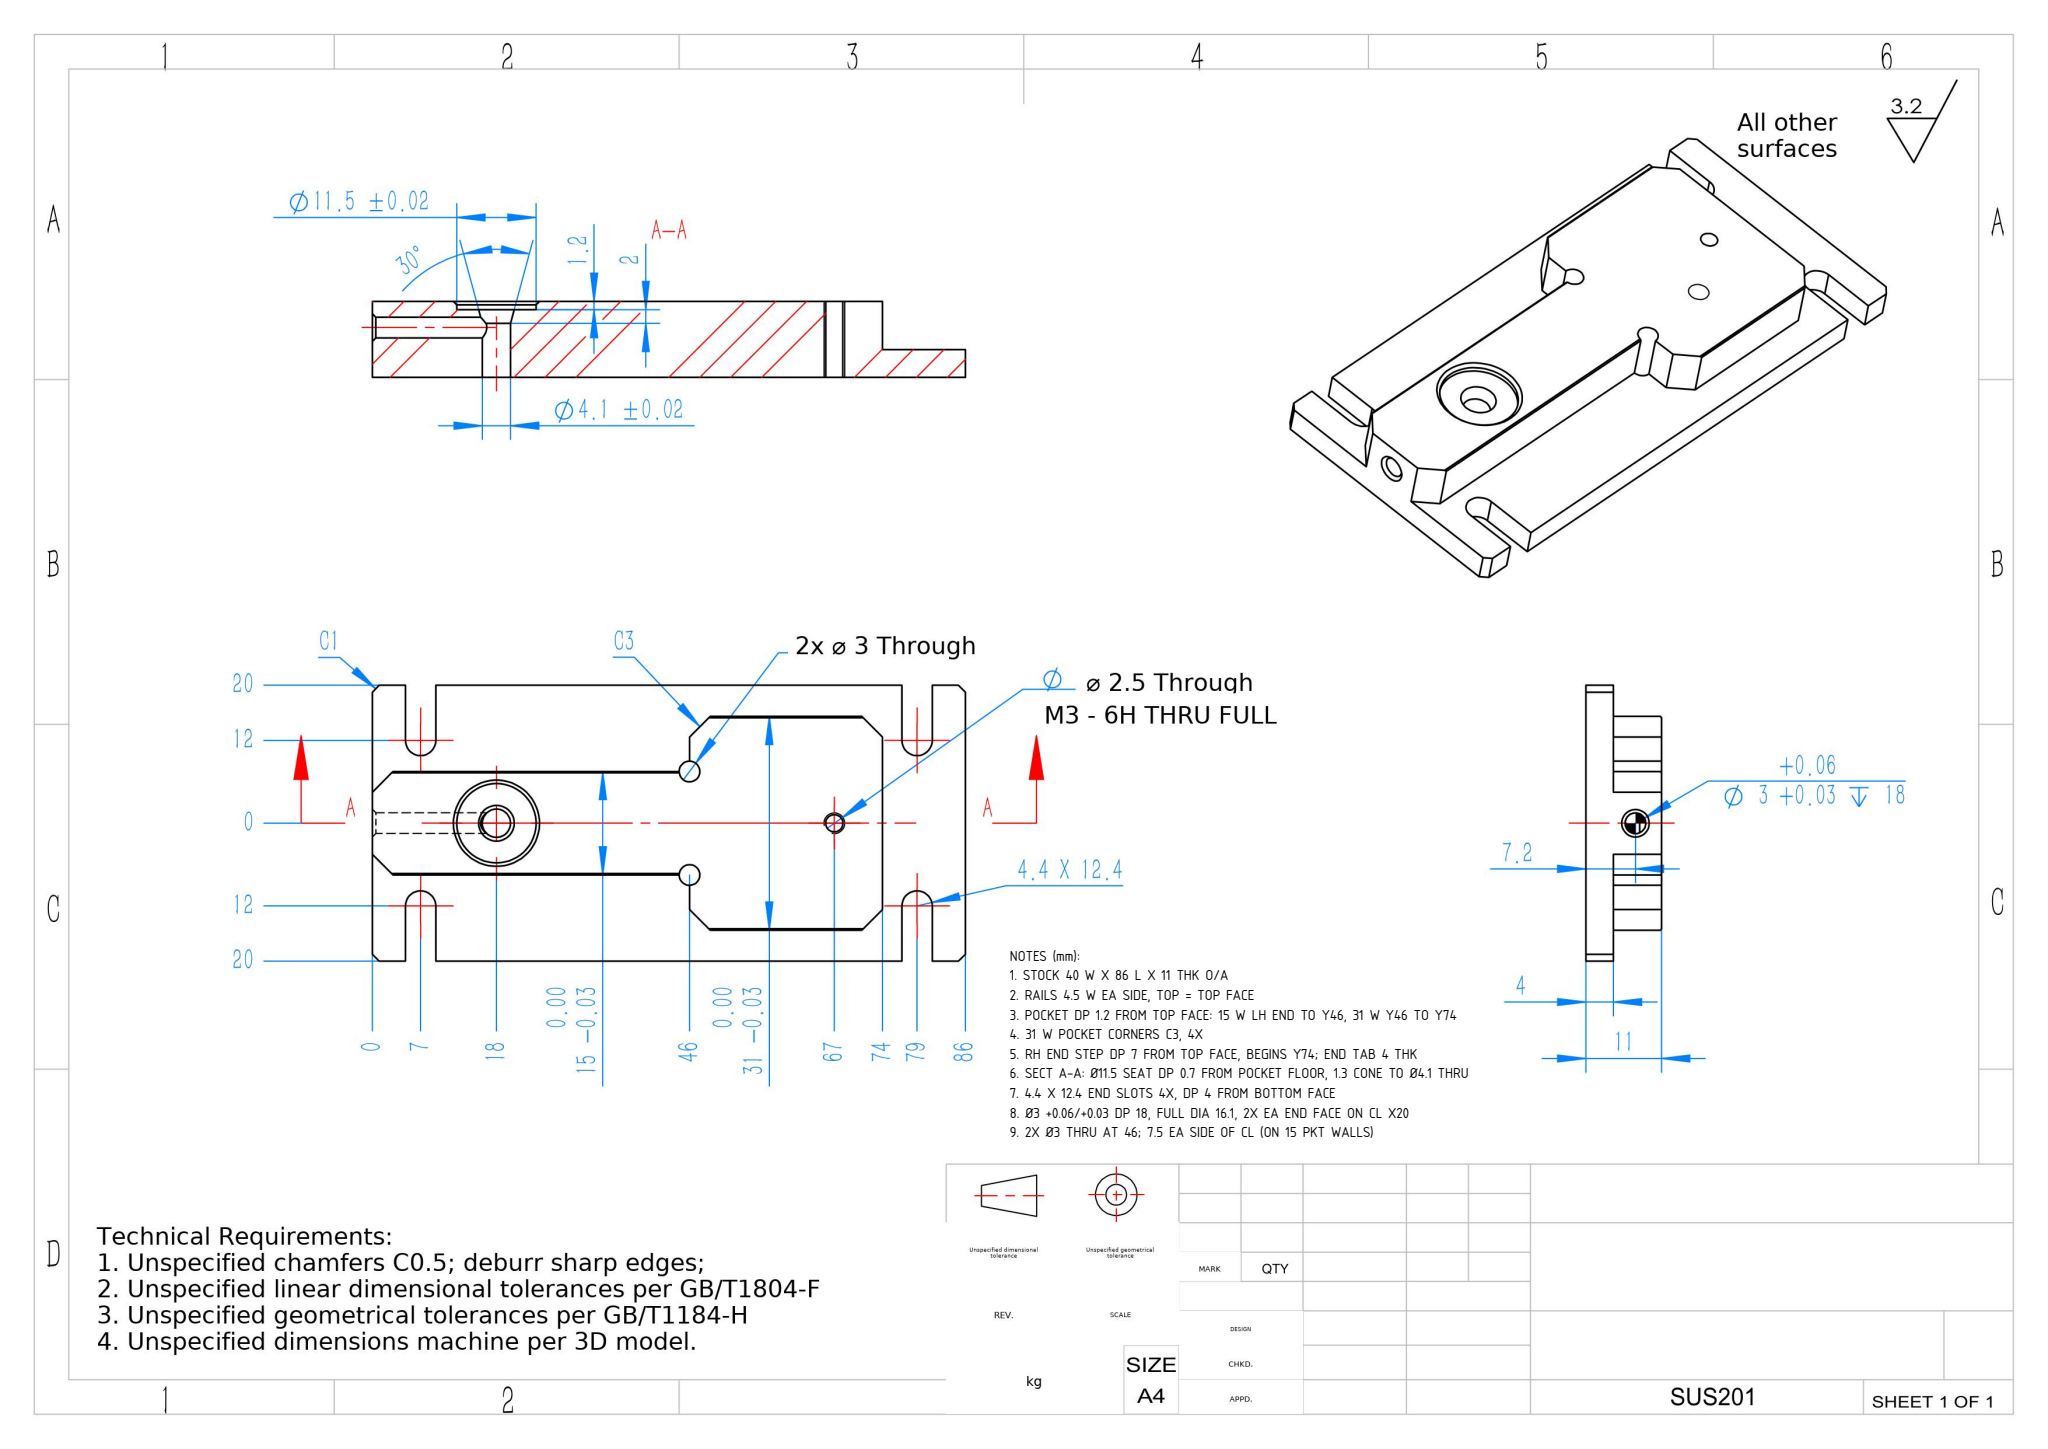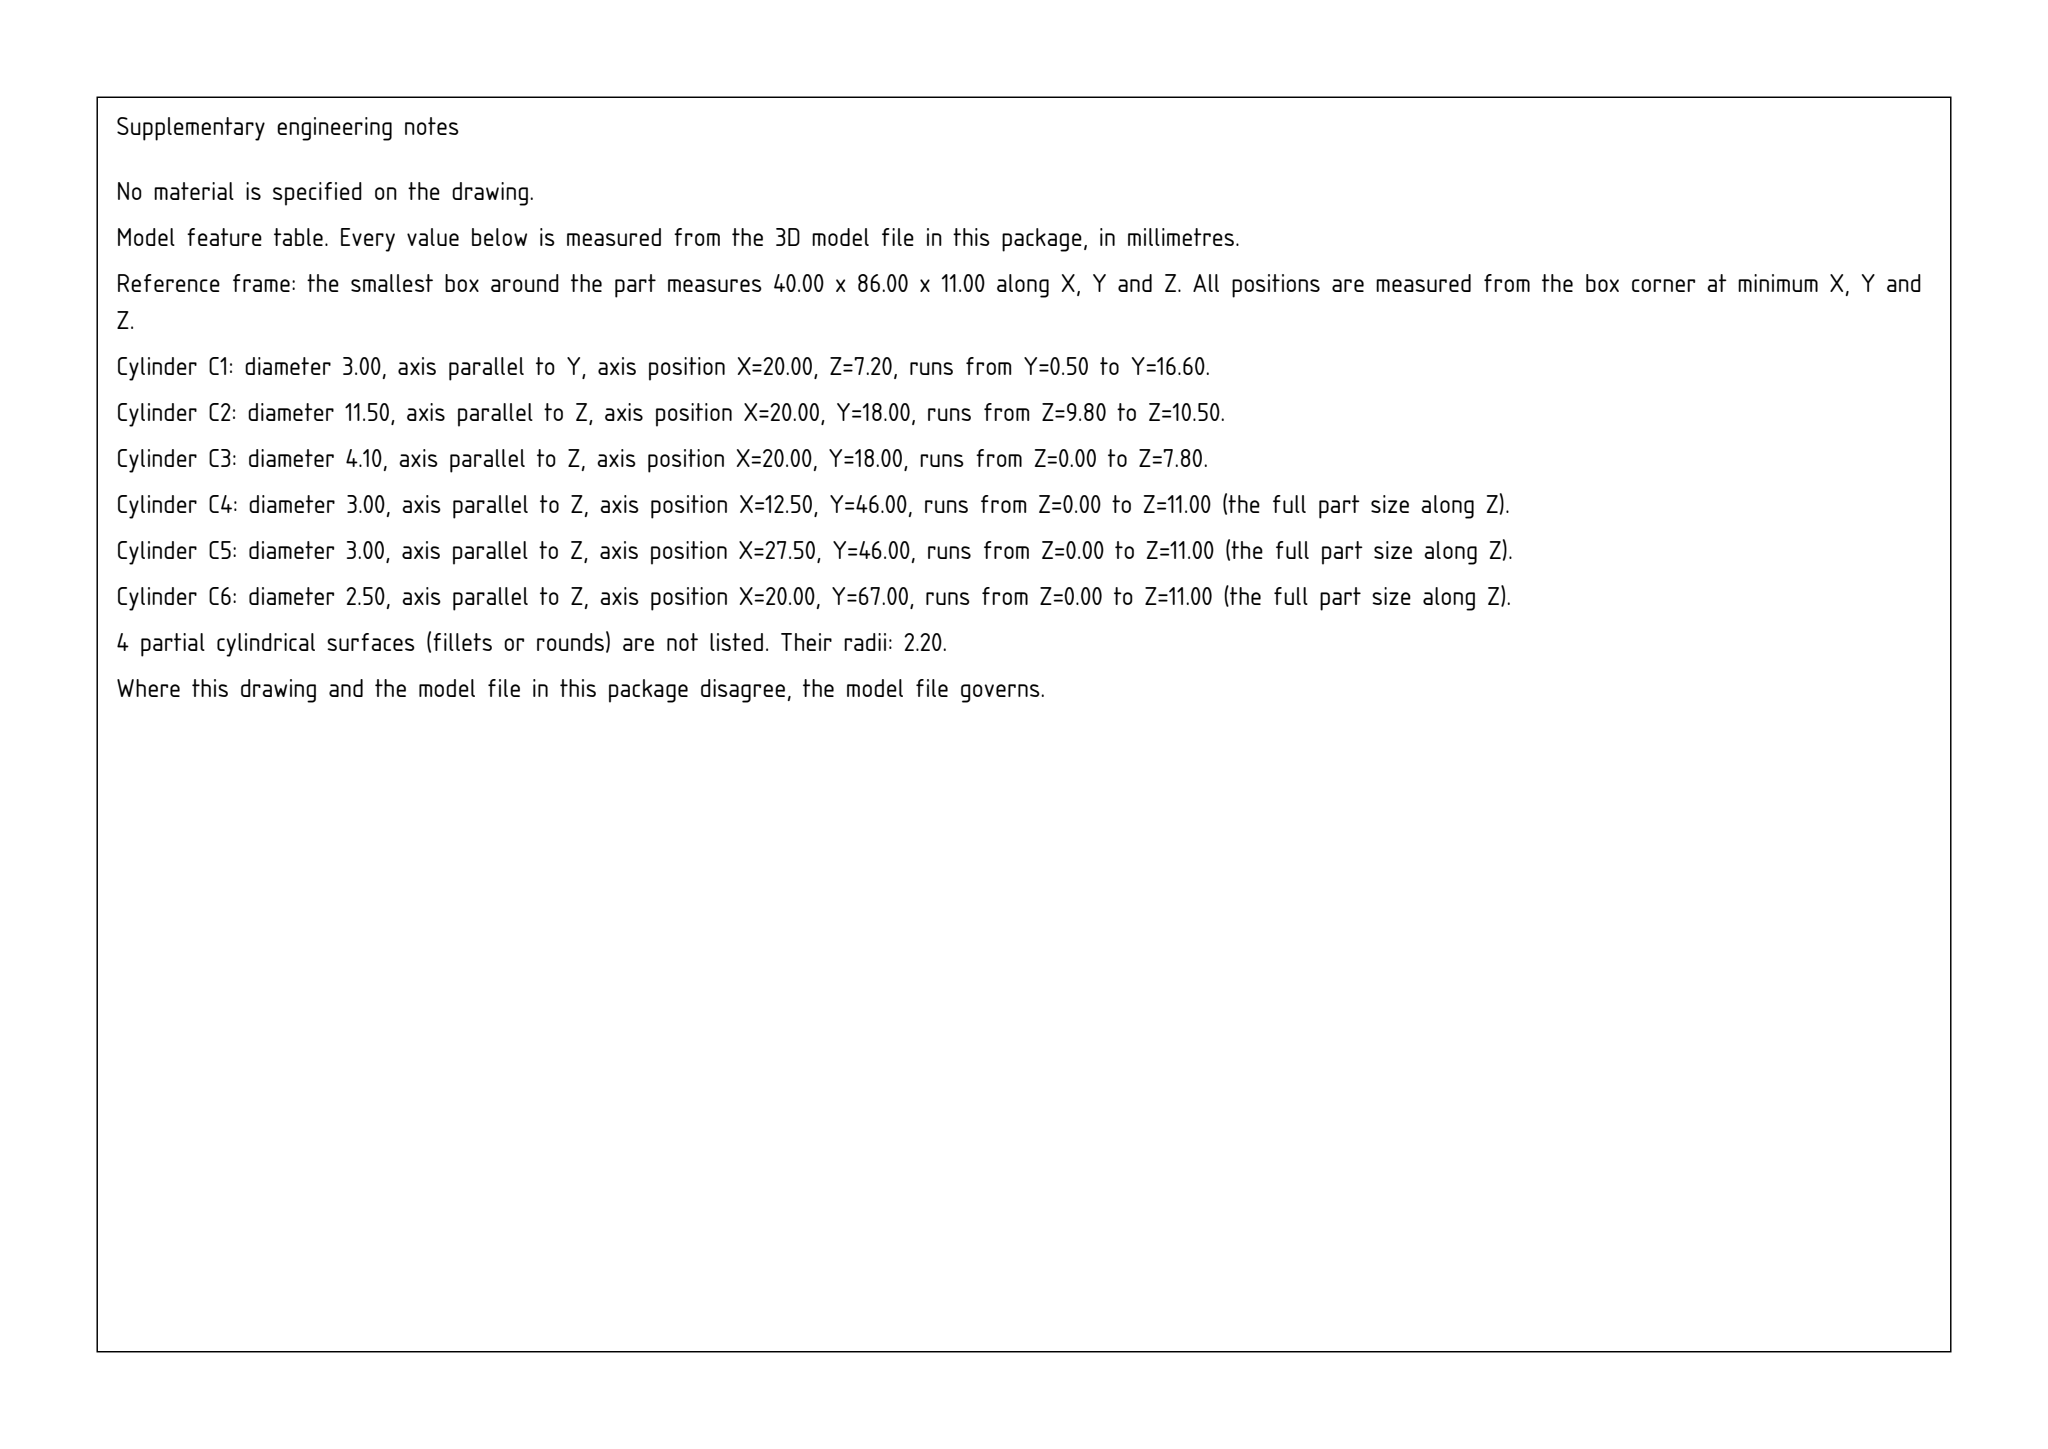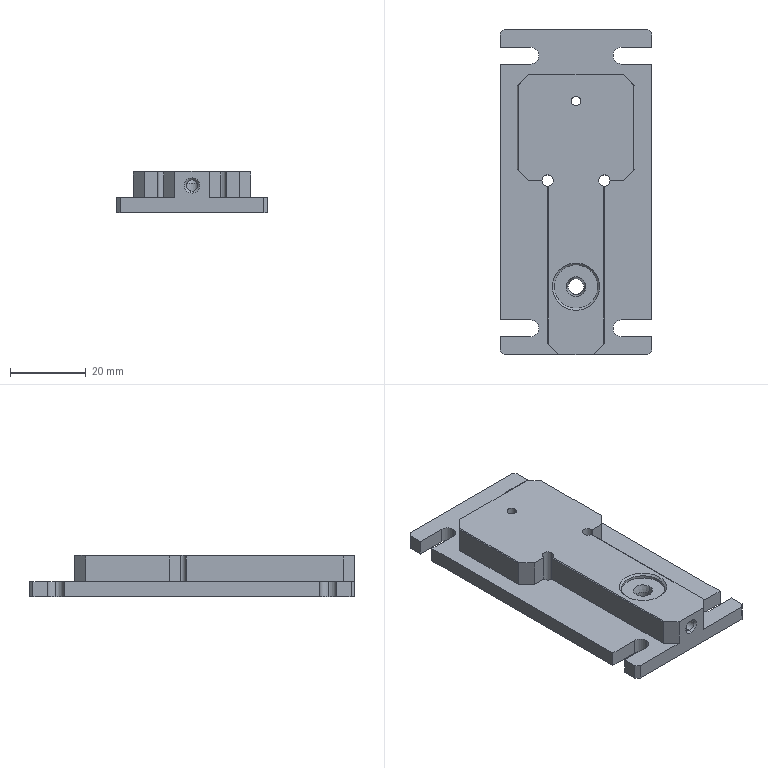Part | SolidWorks | mm | 1 solid | 65 faces | box 40 x 86 x 11 mm | volume 23216 mm3 | plane 41 | cylinder 18 | cone 6 | commonest cylinder face diameters 4.4 x6 3 x6 2.5 x2 4.1 x2 11.5 x2
Drawing notes:
STOCK 40 W X 86 L X 11 THK O/A | from the solid: bbox_xyz 40 x 86 x 11
RAILS 4.5 W EA SIDE, TOP = TOP FACE | from the solid: x-planes 0/4.5 and 35.5/40
POCKET DP 1.2 FROM TOP FACE: 15 W LH END TO Y46, 31 W Y46 TO Y74 | from the solid: z-plane 9.8 vs top 11.0; x 12.5/27.5 (15 W), x 4.5/35.5 (31 W); y 0/46/74
31 W POCKET CORNERS C3, 4X | from the solid: no fillet_radii; 45° corner reliefs at x4.5/35.5, y46/74
RH END STEP DP 7 FROM TOP FACE, BEGINS Y74; END TAB 4 THK | from the solid: y-plane 74.0; step face z=4.0 vs top z=11.0; tab z0-4 to y=86
SECT A-A: Ø11.5 SEAT DP 0.7 FROM POCKET FLOOR, 1.3 CONE TO Ø4.1 THRU | from the solid: Ø11.5 len 0.7 at (20,18); floor z=9.8; Ø4.1 len 7.8 to z=0; 9.8-0.7-7.8=1.3
4.4 X 12.4 END SLOTS 4X, DP 4 FROM BOTTOM FACE | from the solid: Ø4.4 z-cyls at (8,7),(32,7),(8,79),(32,79) len 4.0 from z=0; z-plane 4.0
Ø3 +0.06/+0.03 DP 18, FULL DIA 16.1, 2X EA END FACE ON CL X20 | from the solid: cyl [3.0,'y',x=20,z=7.2,len 16.1,qty 2] + 90° drill point; bbox X=40
2X Ø3 THRU AT 46; 7.5 EA SIDE OF CL (ON 15 PKT WALLS) | from the solid: cylinders dia 3.0 axis z at (12.5,46) and (27.5,46), length 11 = full thk; part CL at x=20, bbox 40x86x11
build123d program:
from build123d import *

# Parameters (mm, degrees)
SKETCH1_W                      = 15
SKETCH1_H                      = 86
BOSS_EXTRUDE1_DEPTH            = 11
SKETCH14_W                     = 40
SKETCH14_H                     = 86
BOSS_EXTRUDE3_DEPTH            = 4
SKETCH3_R                      = 5.75
CUT_EXTRUDE2_DEPTH             = 1.2
F_5_2_5_2_DIAMETER_HOLE1_D     = 4.1
CHAMFER1_SIZE                  = 0.5
CHAMFER2_SIZE                  = 2
CHAMFER2_SIZE2                 = 0.5359
M3_TAPPED_HOLE1_D              = 2.5
SIZE_MM_DOWEL_PIN_HOLE_1_D     = 3
SIZE_MM_DOWEL_PIN_HOLE_1_DEPTH = 18
SIZE_MM_DOWEL_PIN_HOLE_1_TIP   = 0.9013
CHAMFER3_SIZE                  = 0.5
F_4_0_4_DIAMETER_HOLE1_D       = 4
CHAMFER4_SIZE                  = 1
SKETCH19_W                     = 8
SKETCH19_H                     = 28
BOSS_EXTRUDE4_DEPTH            = 7
SKETCH20_W                     = 15
SKETCH20_H                     = 12
CUT_EXTRUDE3_DEPTH             = 48.937
CHAMFER5_SIZE                  = 3
F_3_0_3_DIAMETER_HOLE1_D       = 3
CHAMFER6_SIZE                  = 0.2
CUT_EXTRUDE4_DEPTH             = 49.683


with BuildPart() as part:
    # Sketch1 → Boss-Extrude1 (new body)
    with BuildSketch(Plane.XY):
        Rectangle(SKETCH1_W, SKETCH1_H)
    extrude(amount=BOSS_EXTRUDE1_DEPTH)

    # Sketch14 → Boss-Extrude3 (add)
    with BuildSketch(Plane(origin=(0, 0, 0), x_dir=(-1, 0, 0), z_dir=(0, 0, -1))):
        Rectangle(SKETCH14_W, SKETCH14_H)
    extrude(amount=-BOSS_EXTRUDE3_DEPTH)

    # Sketch3 → Cut-Extrude2 (cut)
    with BuildSketch(Plane.XY.offset(11)):
        with Locations((0, -25)):
            Circle(SKETCH3_R)
    extrude(amount=-CUT_EXTRUDE2_DEPTH, mode=Mode.SUBTRACT)

    # 5.2 _5.2_ Diameter Hole1 (through all)
    with Locations(Plane.XY.offset(9.8)):
        with Locations((0, -25)):
            Hole(F_5_2_5_2_DIAMETER_HOLE1_D / 2)

    # Chamfer1
    chamfer1_edges = [part.edges().sort_by_distance(p)[0] for p in [
        (-5.75, -25, 11),
    ]]
    chamfer(chamfer1_edges, length=CHAMFER1_SIZE)

    # Chamfer2
    chamfer2_edges = [part.edges().sort_by_distance(p)[0] for p in [
        (2.05, -25, 9.8),
    ]]
    chamfer2_side = [part.faces().sort_by_distance(p)[0] for p in [
        (2.05, -25, 4.9),
    ]]
    chamfer(chamfer2_edges, length=CHAMFER2_SIZE, length2=CHAMFER2_SIZE2, reference=chamfer2_side[0])

    # M3 Tapped Hole1 (through all)
    with Locations(Plane(origin=(0, 0, 0), x_dir=(-1, 0, 0), z_dir=(0, 0, -1))):
        with Locations((0, 24)):
            Hole(M3_TAPPED_HOLE1_D / 2)

    # Size mm Dowel Pin Hole 1
    with Locations(Plane(origin=(0, -43, 0), x_dir=(-1, 0, 0), z_dir=(0, -1, 0))):
        with Locations((0, -7.2)):
            Hole(SIZE_MM_DOWEL_PIN_HOLE_1_D / 2, depth=SIZE_MM_DOWEL_PIN_HOLE_1_DEPTH)
            with Locations((0, 0, -(SIZE_MM_DOWEL_PIN_HOLE_1_DEPTH + SIZE_MM_DOWEL_PIN_HOLE_1_TIP / 2))):  # 118° drill point
                Cone(0, SIZE_MM_DOWEL_PIN_HOLE_1_D / 2, SIZE_MM_DOWEL_PIN_HOLE_1_TIP, mode=Mode.SUBTRACT)

    # Chamfer3
    chamfer3_edges = [part.edges().sort_by_distance(p)[0] for p in [
        (-1.5, -43, 7.2),
    ]]
    chamfer(chamfer3_edges, length=CHAMFER3_SIZE)

    # 4.0 _4_ Diameter Hole1 (through all)
    with Locations(Plane.XY.offset(4)):
        with Locations((15, 36), (-15, 36), (-15, -36), (15, -36)):
            Hole(F_4_0_4_DIAMETER_HOLE1_D / 2)

    # Chamfer4
    chamfer4_edges = [part.edges().sort_by_distance(p)[0] for p in [
        (-20, -43, 2),
        (20, 43, 2),
        (-20, 43, 2),
        (20, -43, 2),
    ]]
    chamfer(chamfer4_edges, length=CHAMFER4_SIZE)

    # Sketch19 → Boss-Extrude4 (add)
    with BuildSketch(Plane.XY.offset(4)):
        with Locations((-11.5, 17)):
            Rectangle(SKETCH19_W, SKETCH19_H)
        with Locations((11.5, 17)):
            Rectangle(SKETCH19_W, SKETCH19_H)
    extrude(amount=BOSS_EXTRUDE4_DEPTH)

    # Sketch20 → Cut-Extrude3 (cut, through all)
    with BuildSketch(Plane.XY.offset(4)):
        with Locations((0, 37)):
            Rectangle(SKETCH20_W, SKETCH20_H)
    extrude(amount=CUT_EXTRUDE3_DEPTH, mode=Mode.SUBTRACT)

    # Chamfer5
    chamfer5_edges = [part.edges().sort_by_distance(p)[0] for p in [
        (-15.5, 31, 7.5),
        (-15.5, 3, 7.5),
        (15.5, 31, 7.5),
        (15.5, 3, 7.5),
        (7.5, -43, 7.5),
        (-7.5, -43, 7.5),
    ]]
    chamfer(chamfer5_edges, length=CHAMFER5_SIZE)

    # 3.0 _3_ Diameter Hole1 (through all)
    with Locations(Plane.XY.offset(11)):
        with Locations((-7.5, 3), (7.5, 3)):
            Hole(F_3_0_3_DIAMETER_HOLE1_D / 2)

    # Chamfer6
    chamfer6_edges = [part.edges().sort_by_distance(p)[0] for p in [
        (15.5, 17, 11),
        (-15.5, 17, 11),
        (7.5, -19.25, 11),
        (-7.5, -19.25, 11),
    ]]
    chamfer(chamfer6_edges, length=CHAMFER6_SIZE)

    # Sketch21 → Cut-Extrude4 (cut, through all)
    with BuildSketch(Plane.XY.offset(11)):
        with BuildLine():
            Line((12, 38.2), (20, 38.2))
            ThreePointArc((20, 38.2), (22.2, 36), (20, 33.8))
            Line((20, 33.8), (12, 33.8))
            ThreePointArc((12, 33.8), (9.8, 36), (12, 38.2))
        make_face()
        with BuildLine():
            Line((12, -38.2), (20, -38.2))
            ThreePointArc((20, -38.2), (22.2, -36), (20, -33.8))
            Line((20, -33.8), (12, -33.8))
            ThreePointArc((12, -33.8), (9.8, -36), (12, -38.2))
        make_face()
        with BuildLine():
            Line((-12, -38.2), (-20, -38.2))
            ThreePointArc((-20, -38.2), (-22.2, -36), (-20, -33.8))
            Line((-20, -33.8), (-12, -33.8))
            ThreePointArc((-12, -33.8), (-9.8, -36), (-12, -38.2))
        make_face()
        with BuildLine():
            Line((-12, 38.2), (-20, 38.2))
            ThreePointArc((-20, 38.2), (-22.2, 36), (-20, 33.8))
            Line((-20, 33.8), (-12, 33.8))
            ThreePointArc((-12, 33.8), (-9.8, 36), (-12, 38.2))
        make_face()
    extrude(amount=-CUT_EXTRUDE4_DEPTH, mode=Mode.SUBTRACT)


solid = part.part